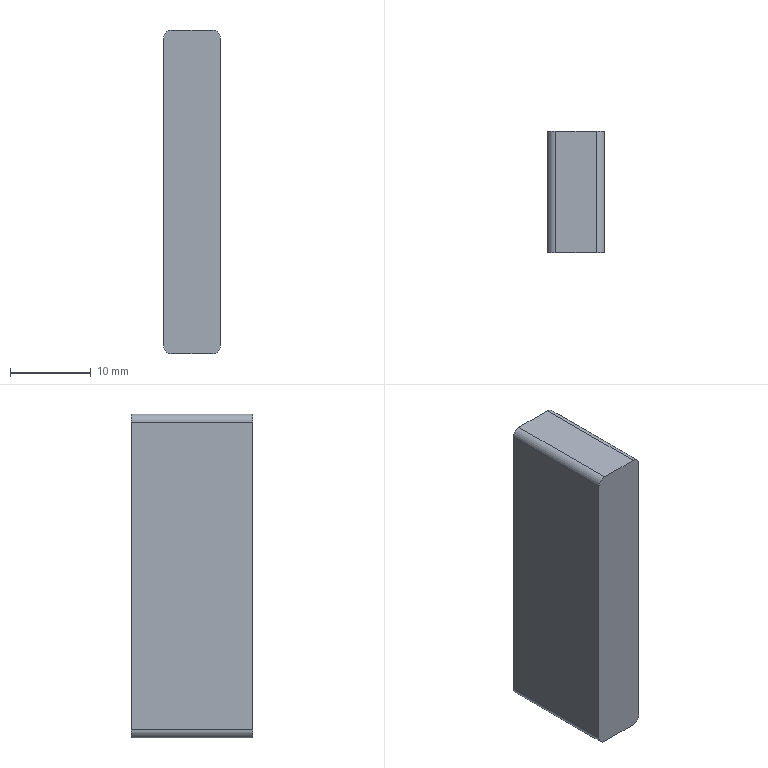CAM job | Mastercam | mm | 7 operations | part box 7 x 15 x 40
1. Facing | 12 - 12 平铣刀
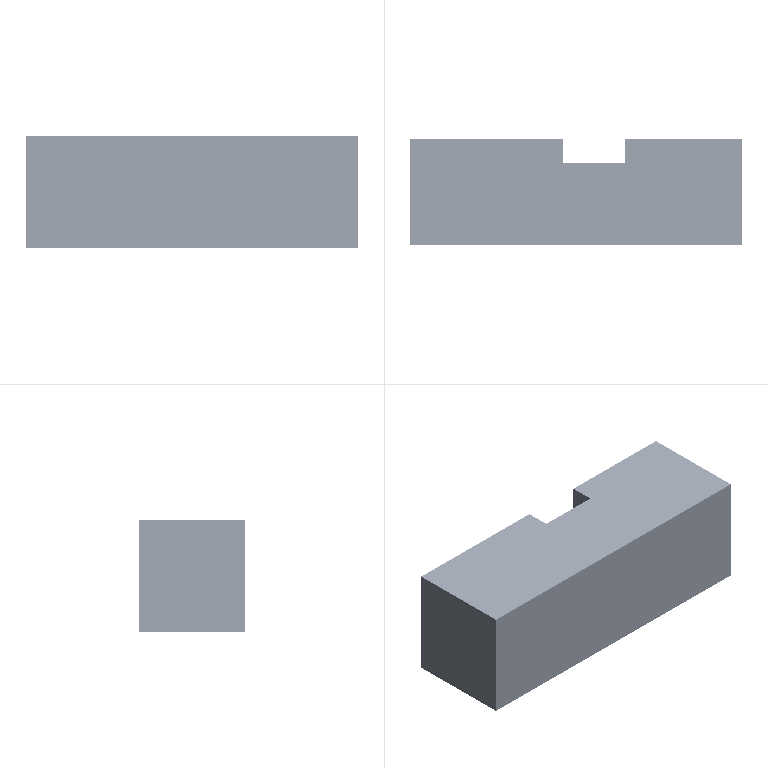2. Contour (Ramp) | 12 - 12 平铣刀
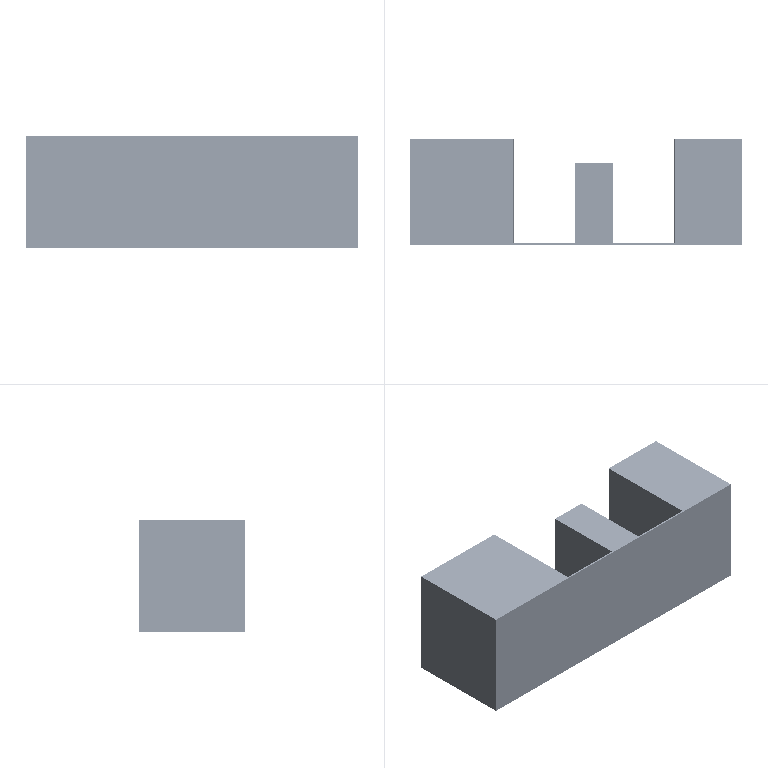3. Contour (2D) | 12 - 12 平铣刀
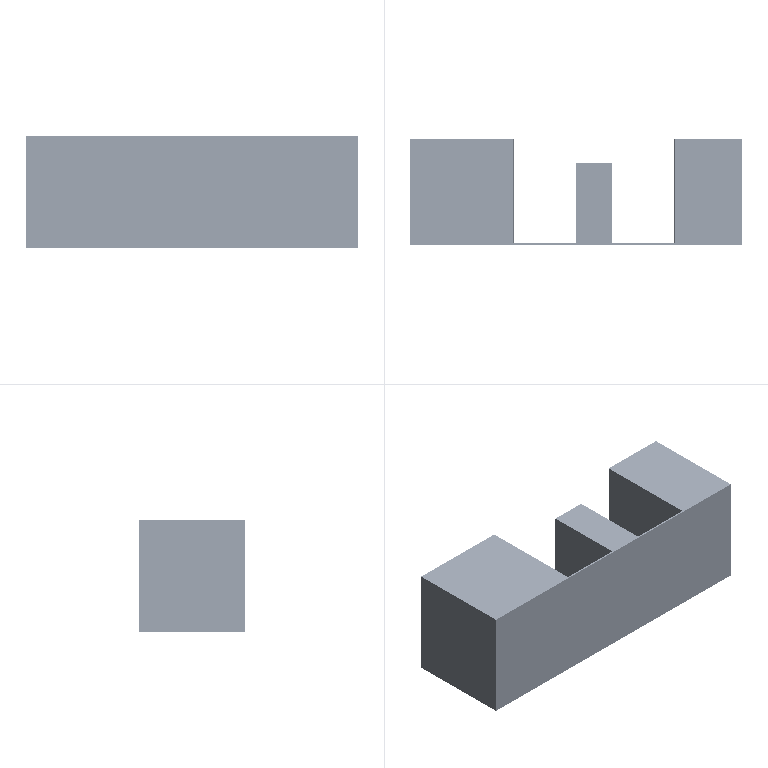4. Contour (2D chamfer) | 7 - 4 倒角刀
5. Drill/Counterbore | 7 - 4 倒角刀
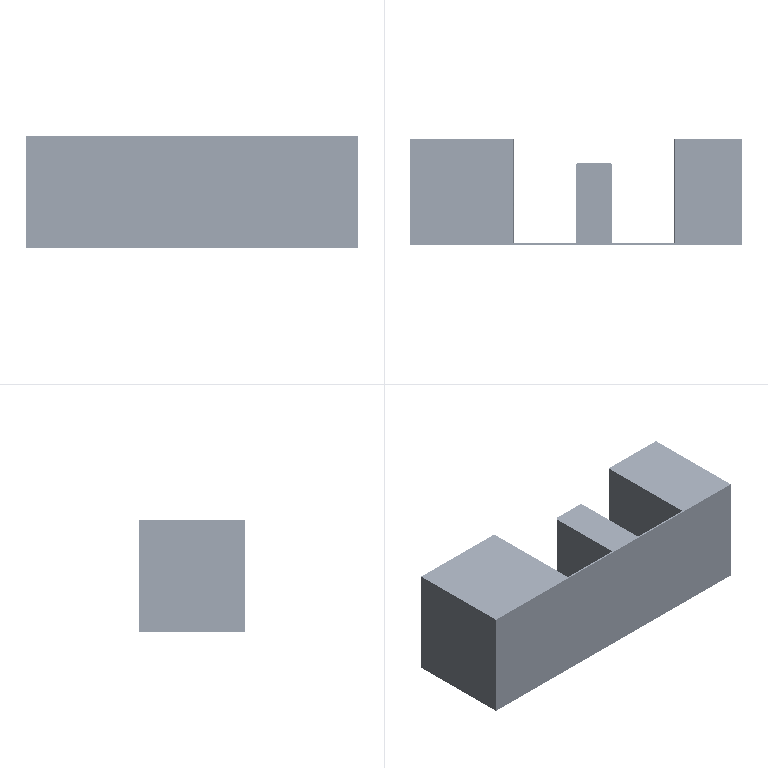6. Facing | 12 - 12 平铣刀
7. Contour (2D chamfer) | 7 - 4 倒角刀